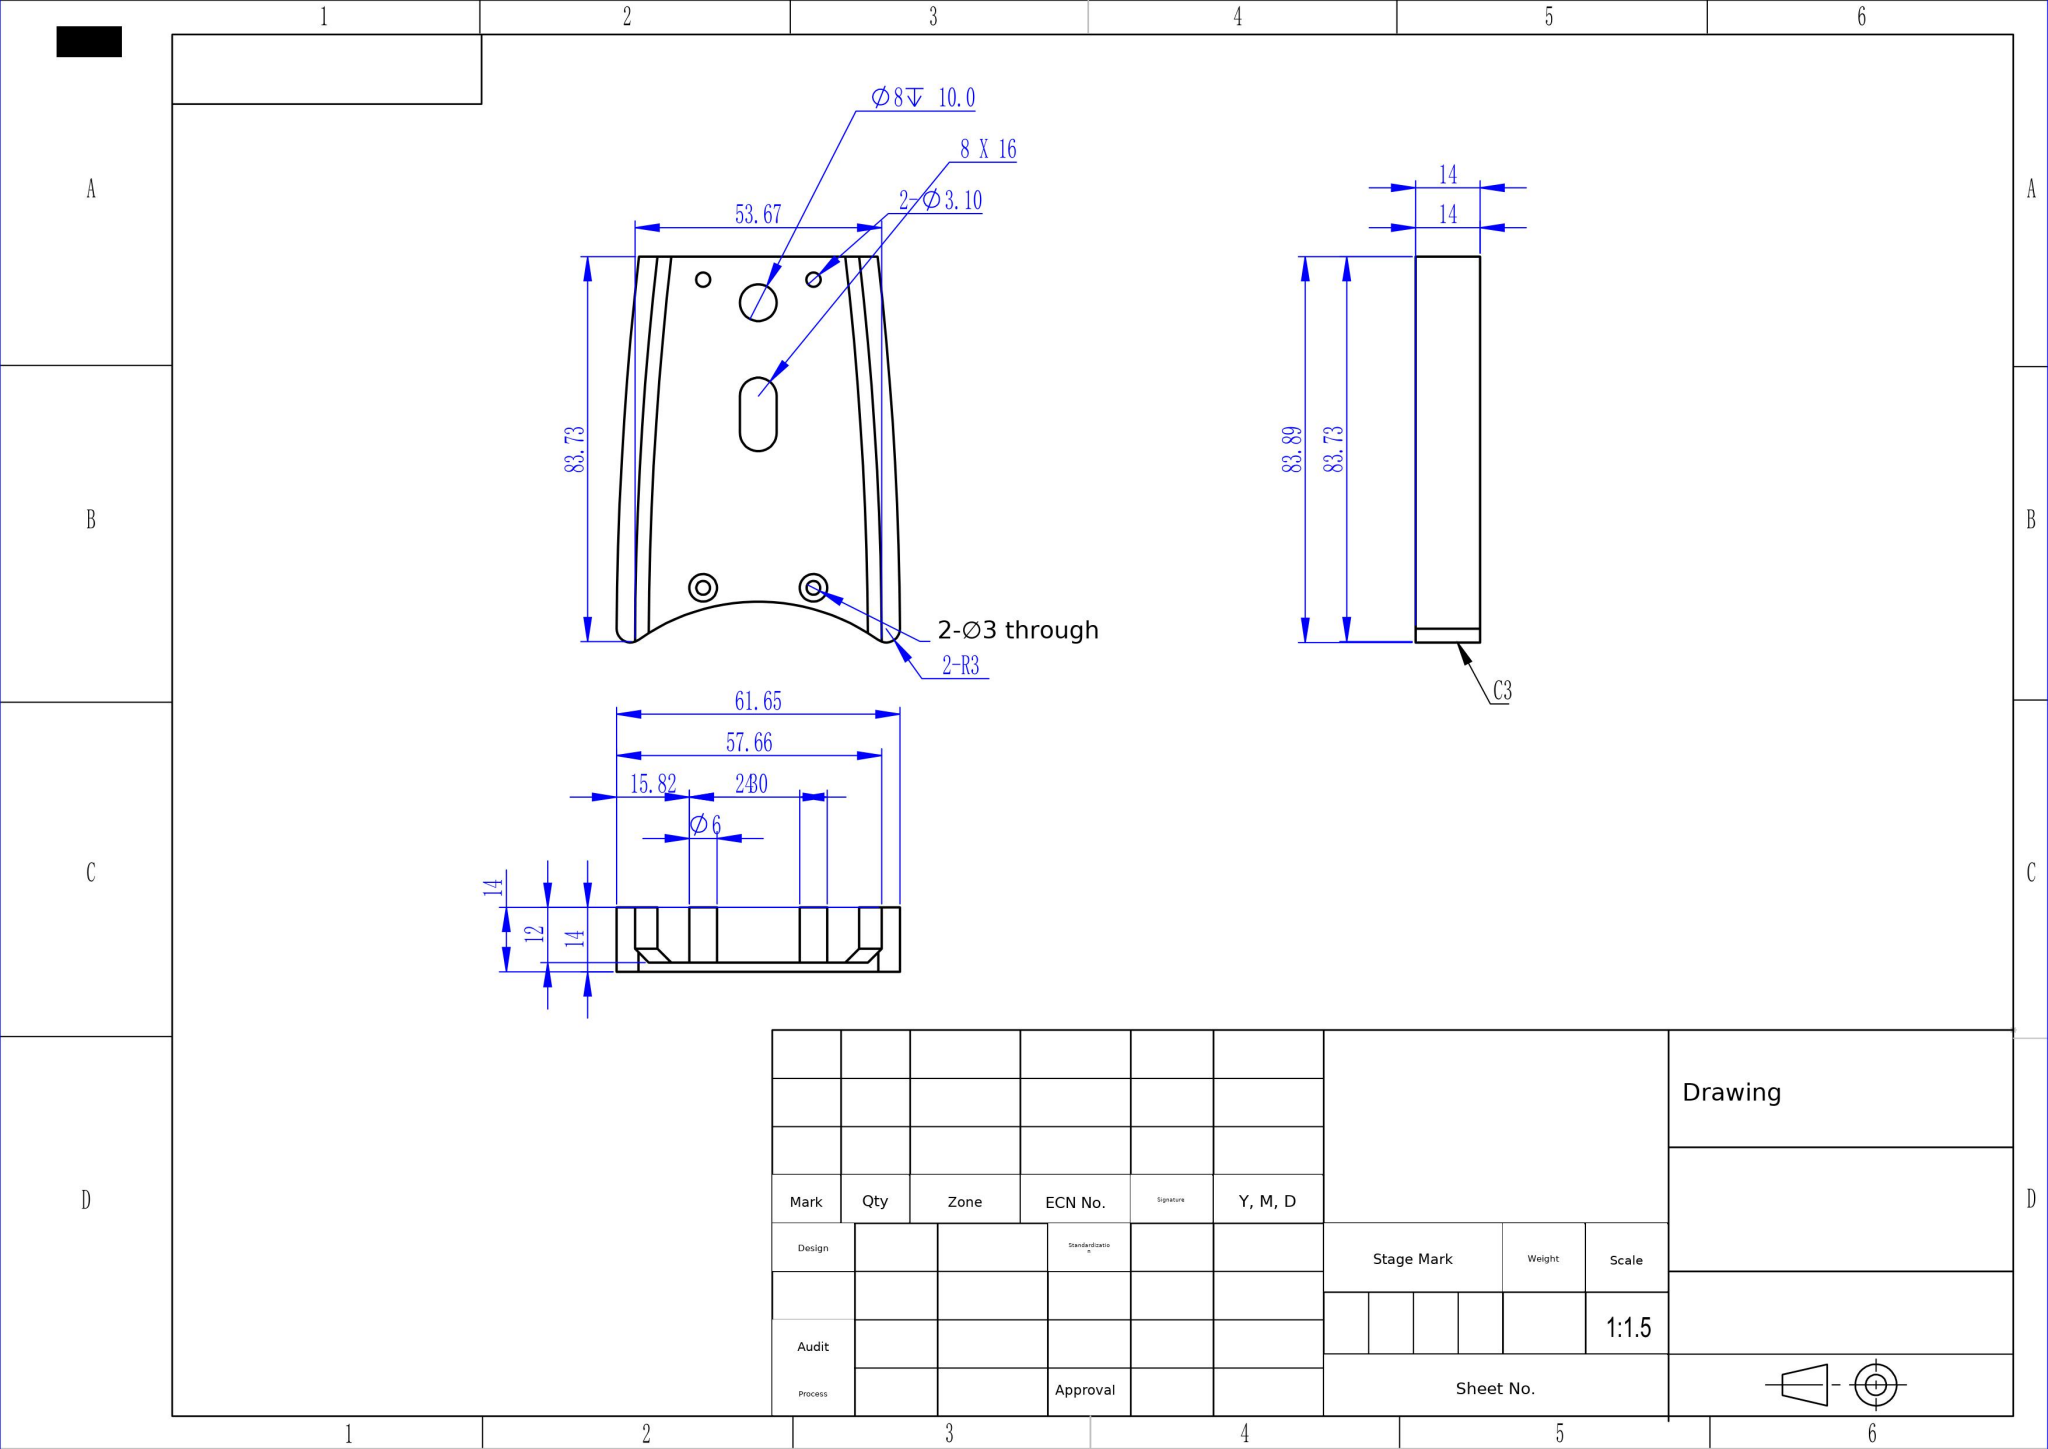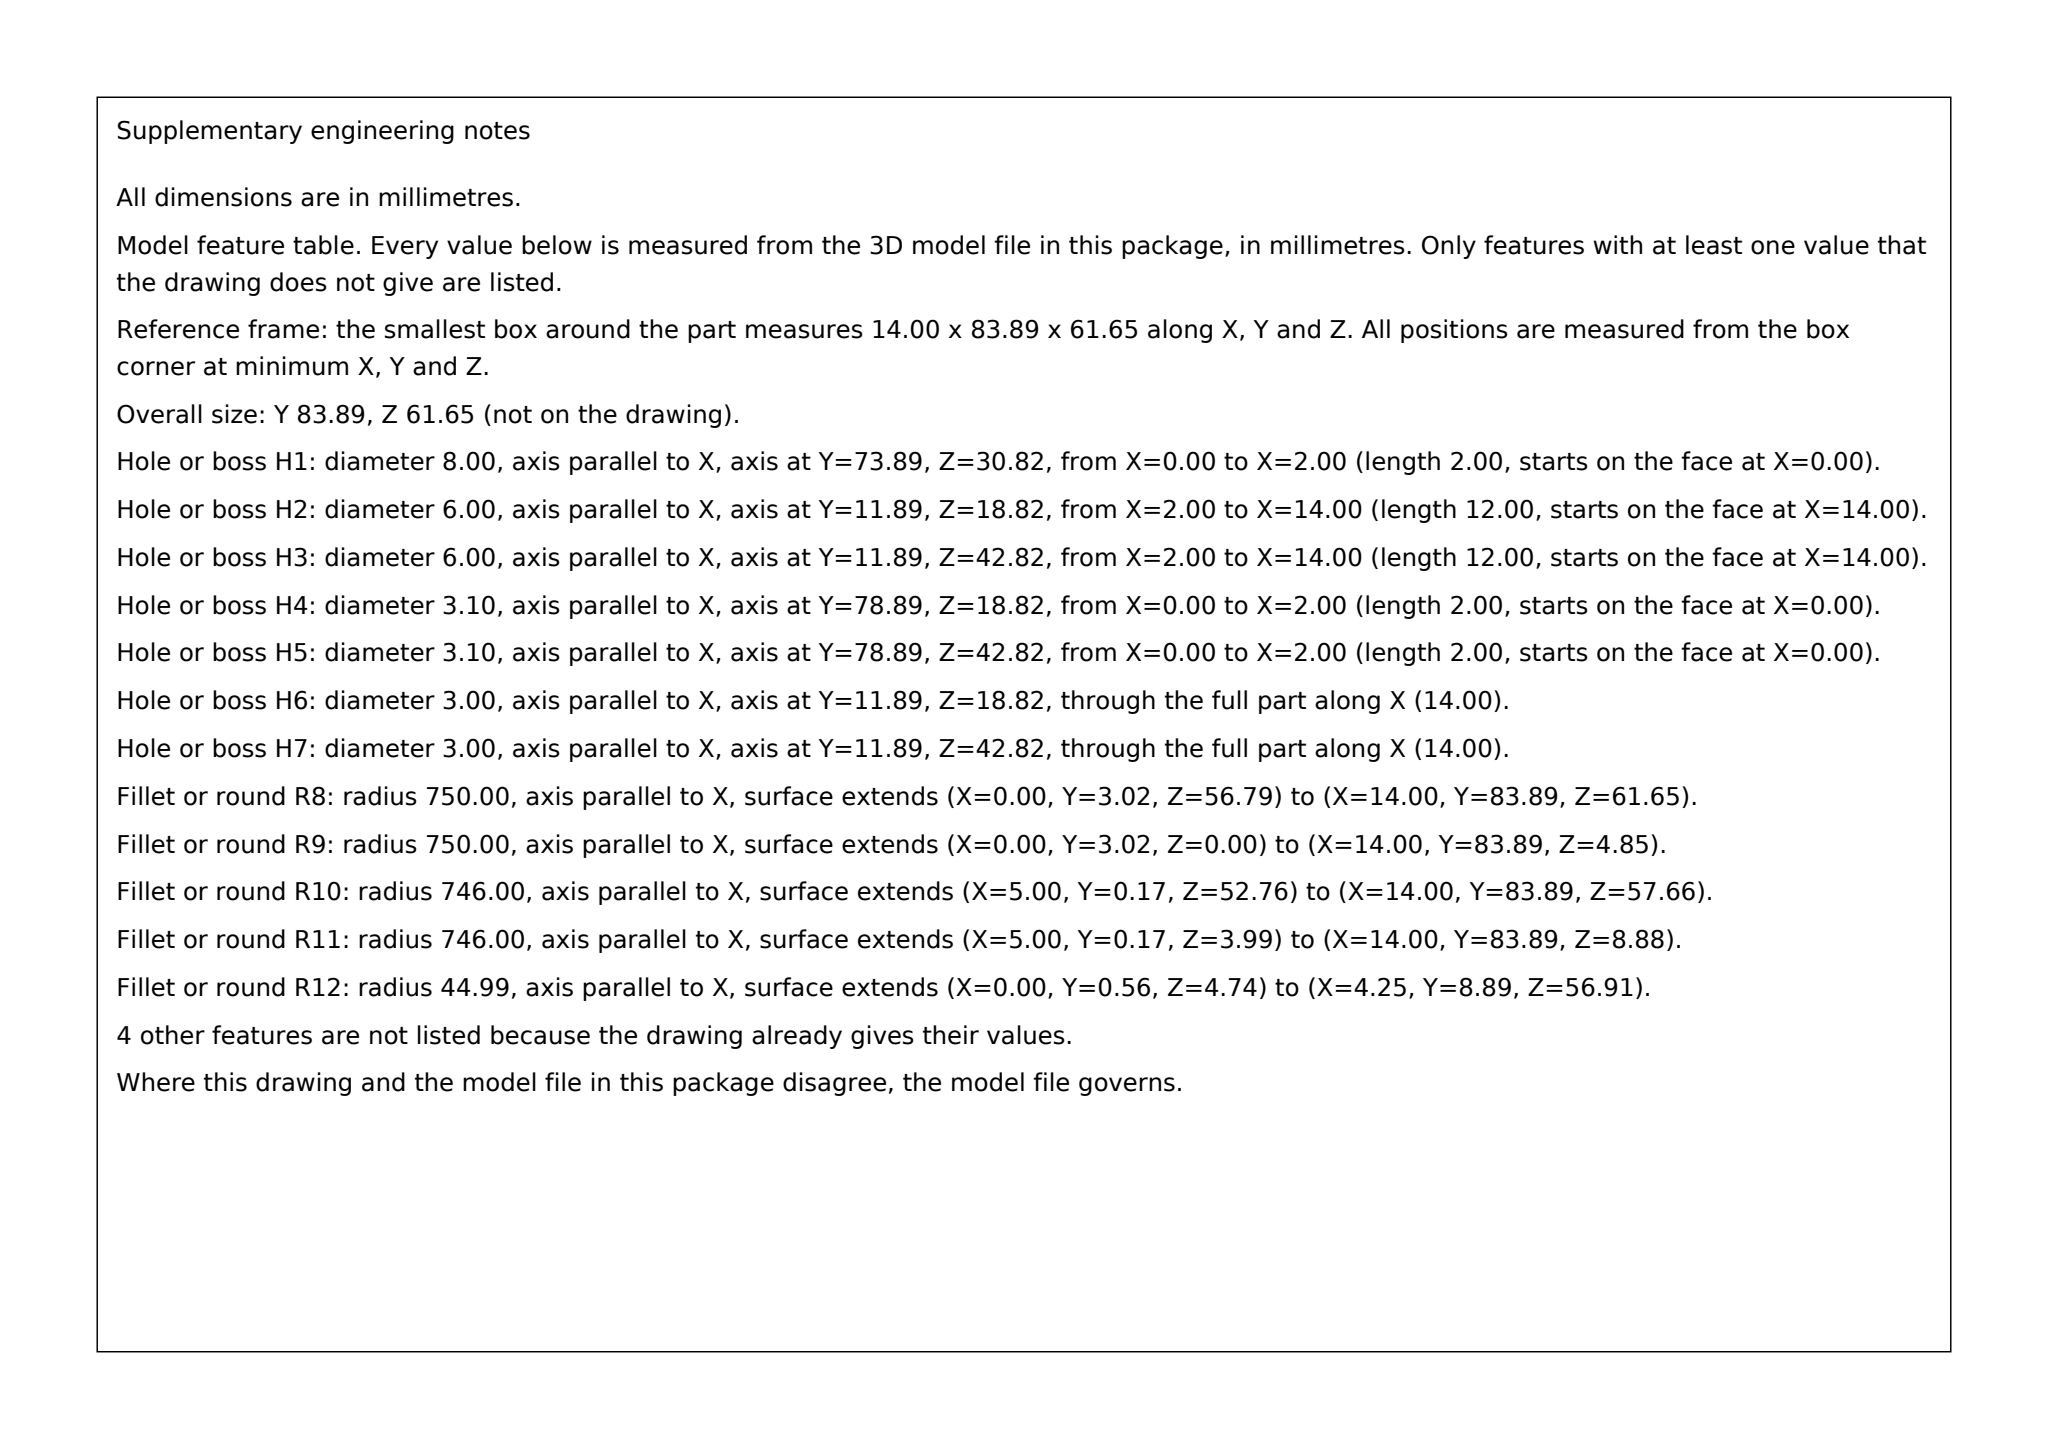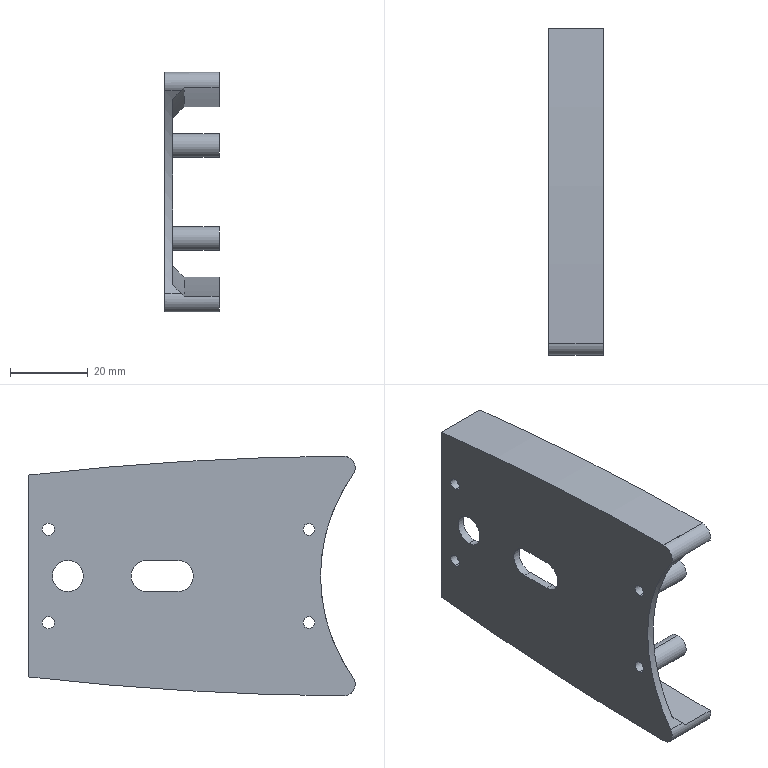Part | SolidWorks | mm | 1 solid | 35 faces | box 14 x 83.89 x 61.65 mm | volume 18031 mm3 | cylinder 24 | plane 9 | cone 2 | commonest cylinder face diameters 6 x7 8 x4 3 x4 3.1 x4 1500 x2 1492 x2 89.989 x1